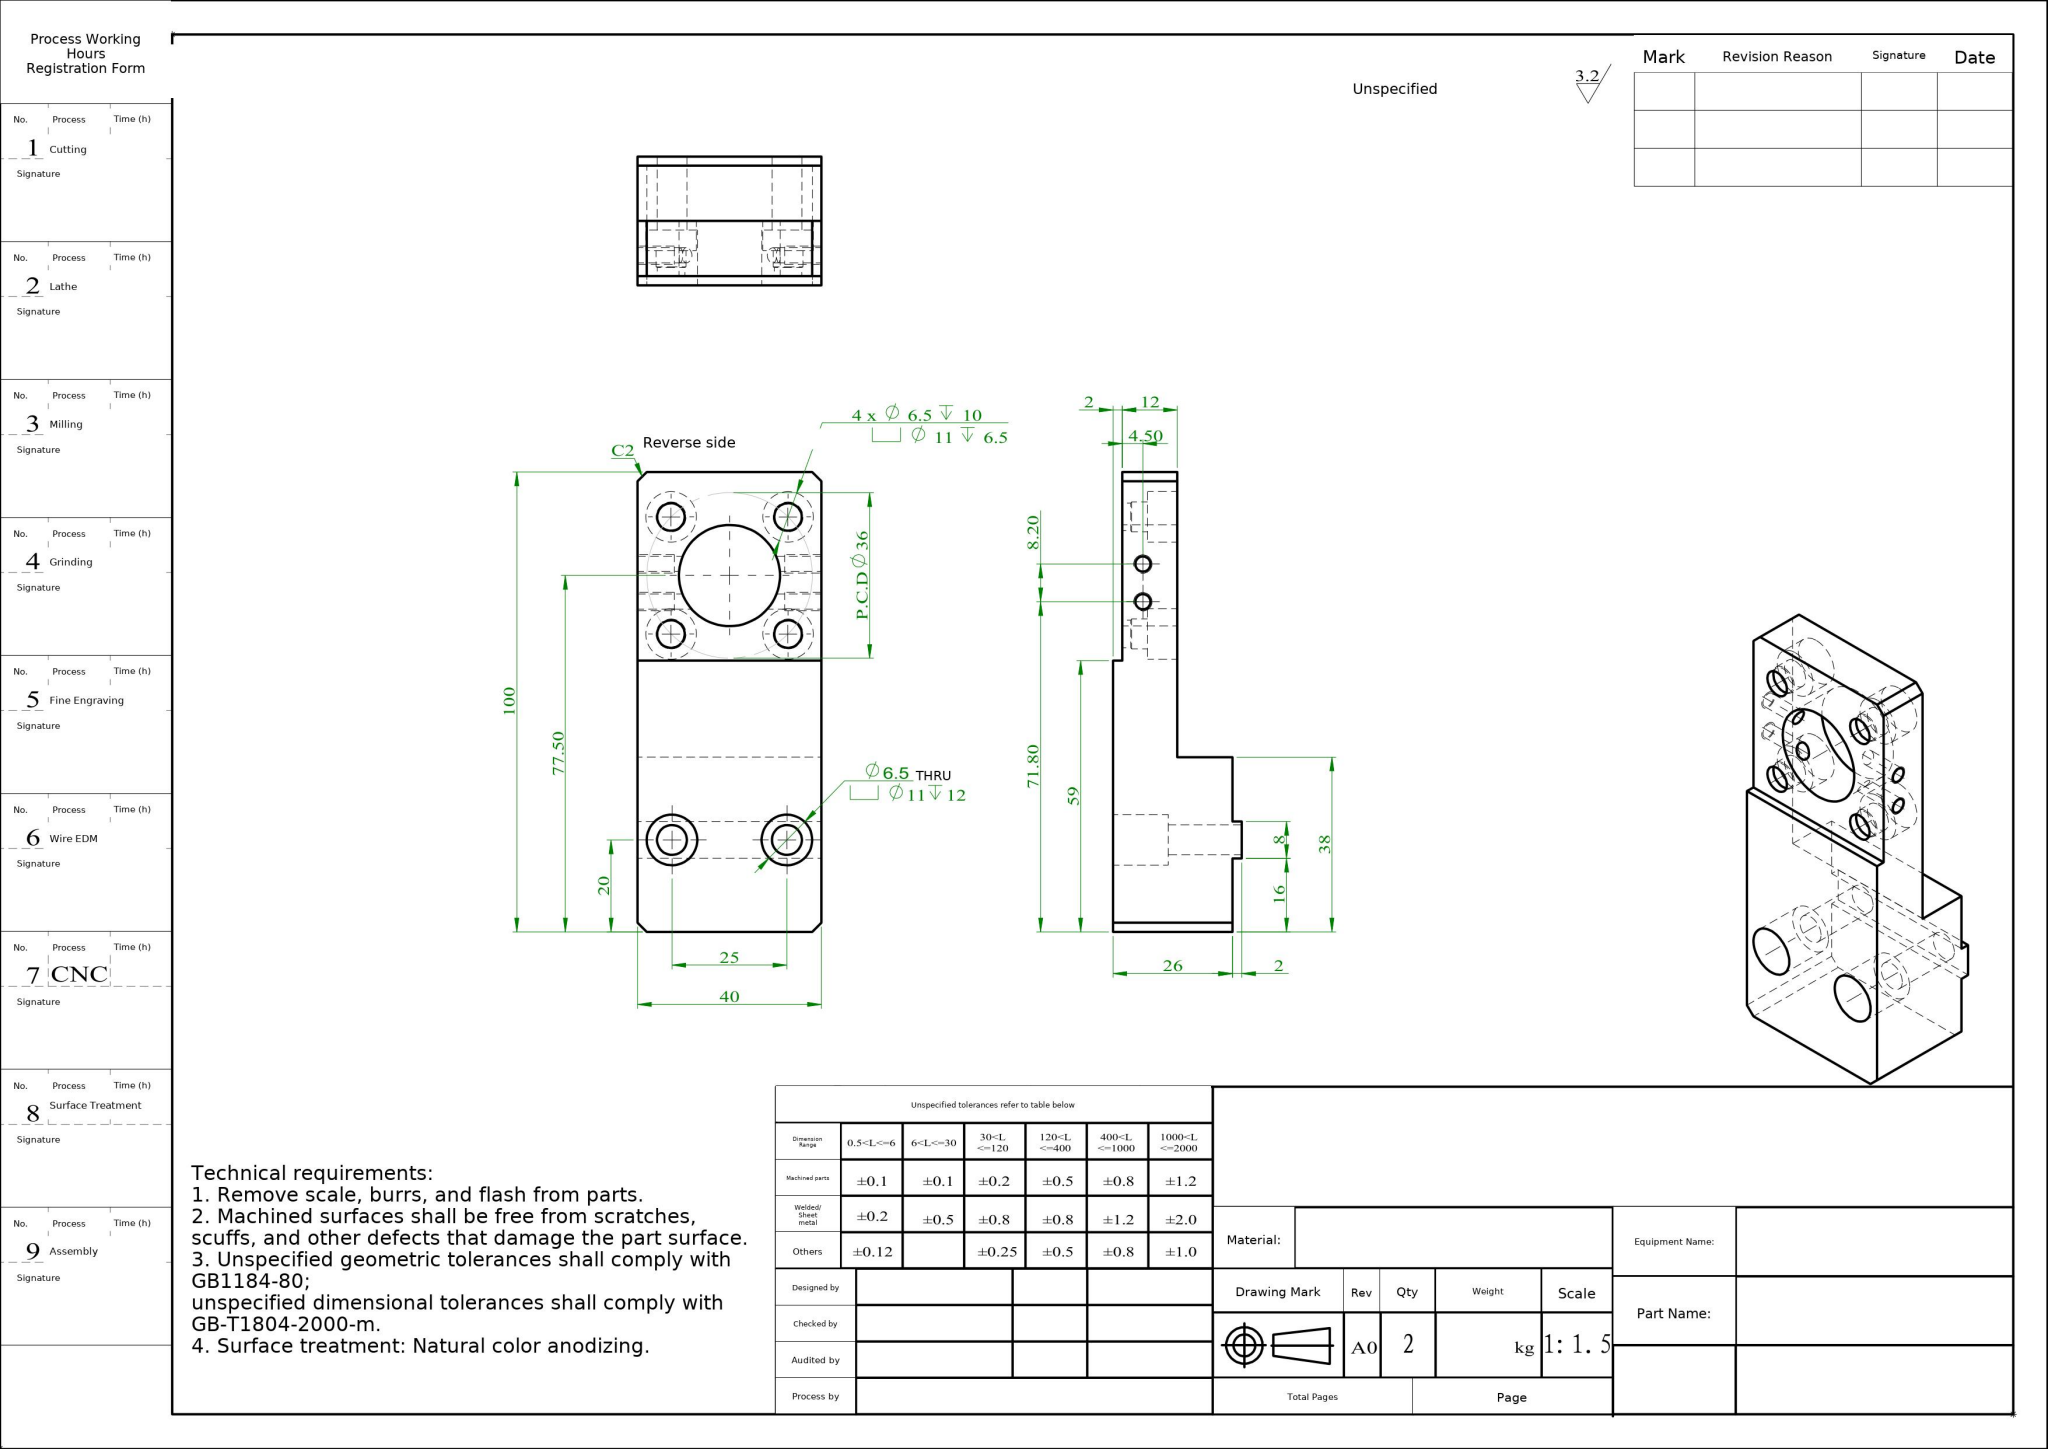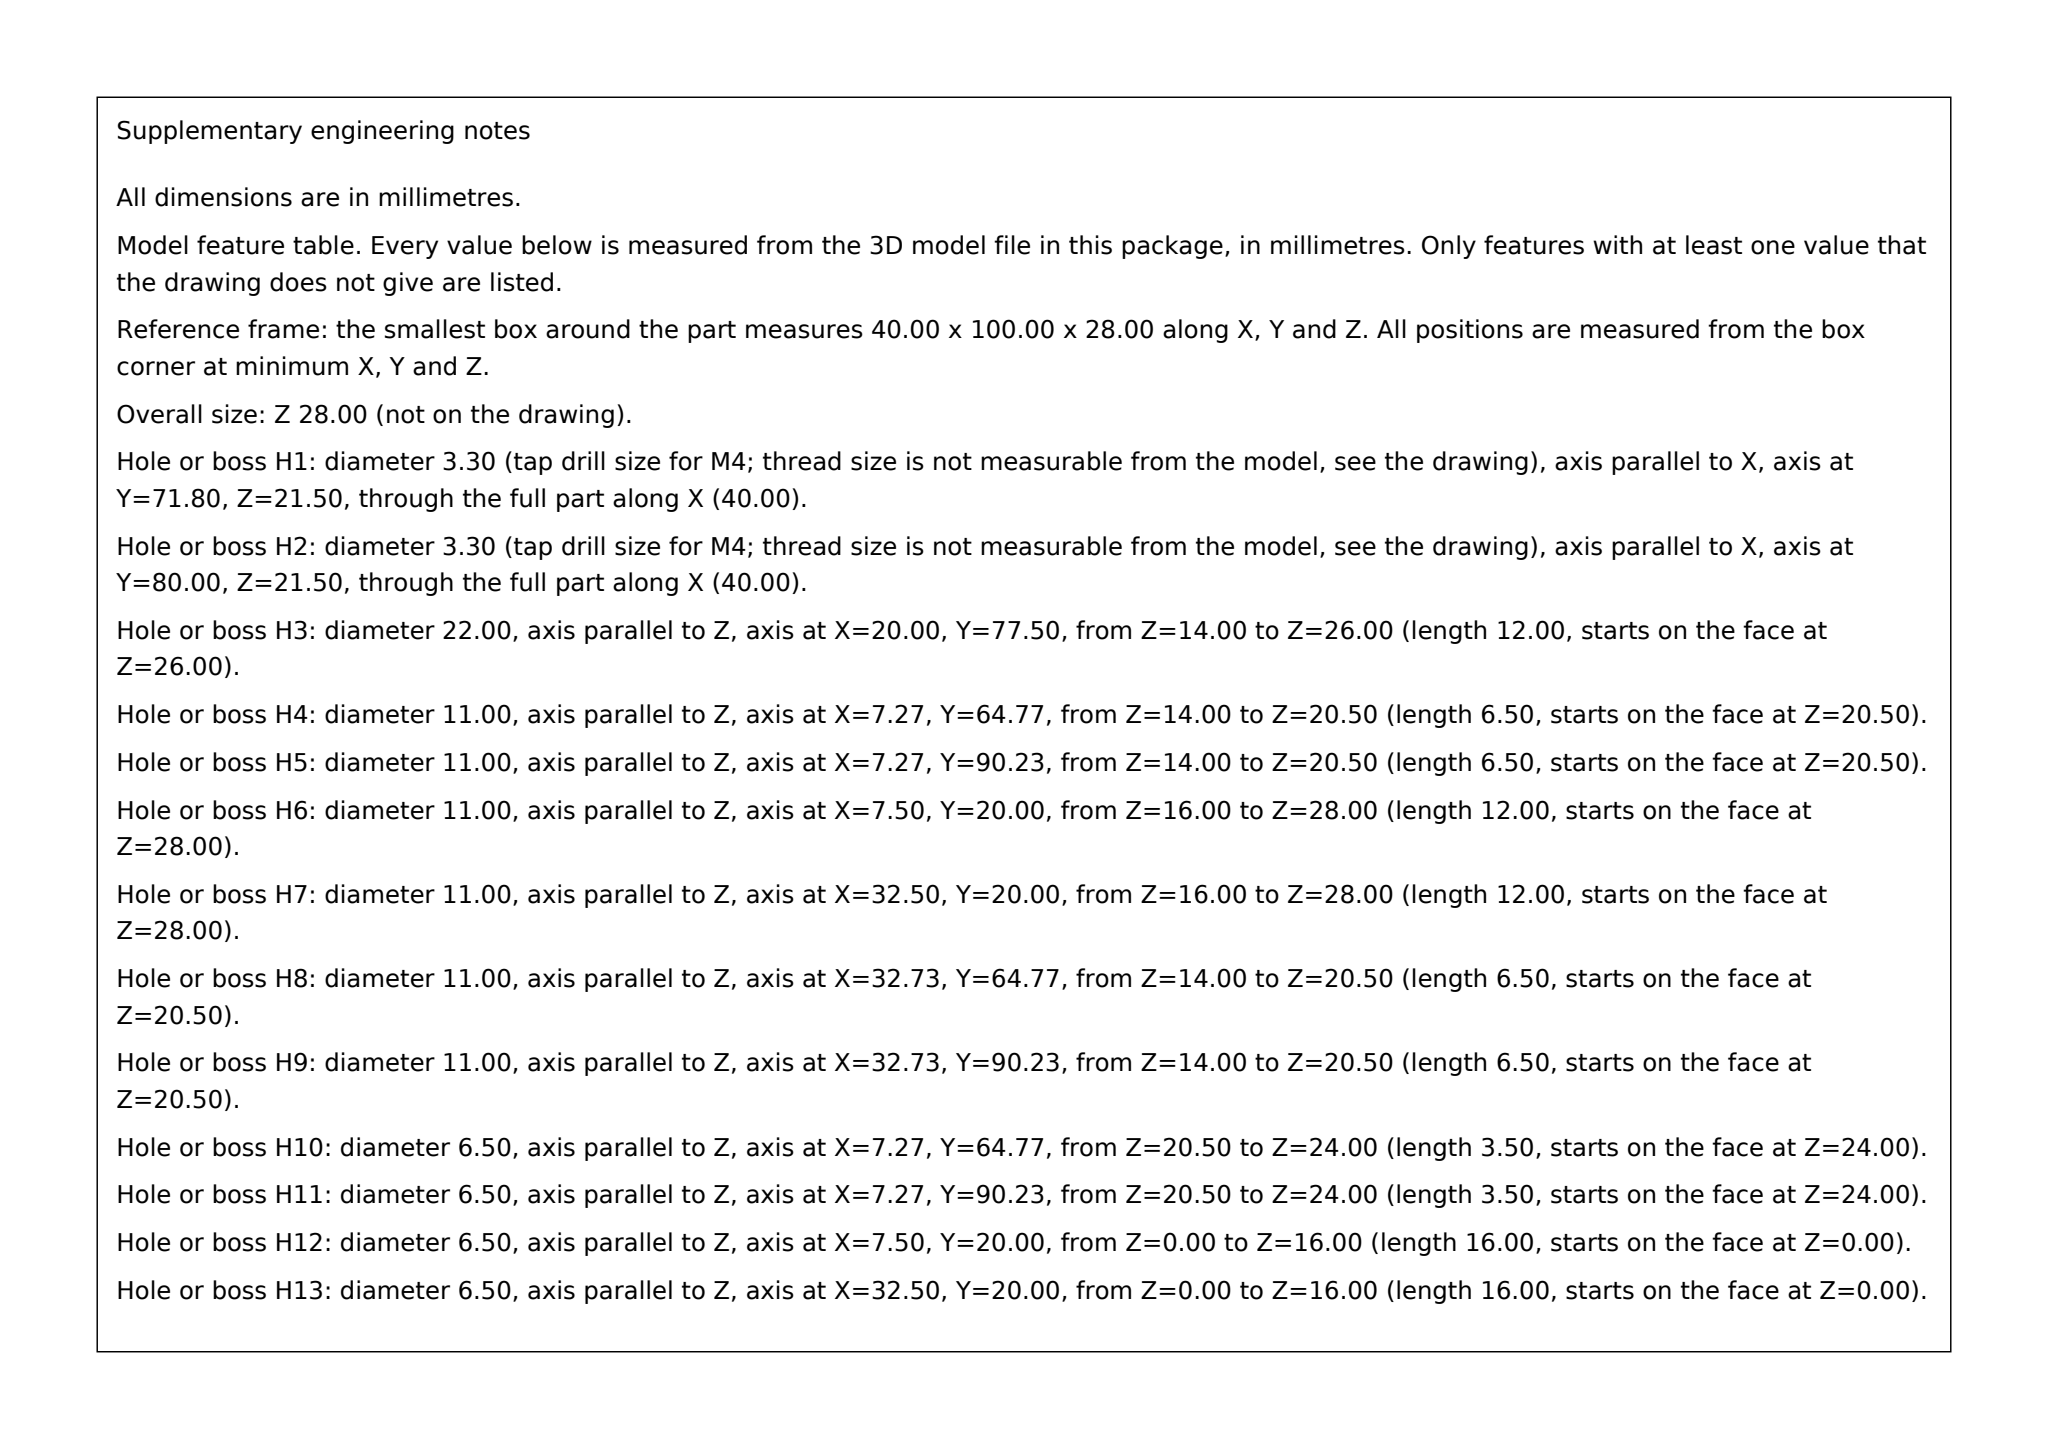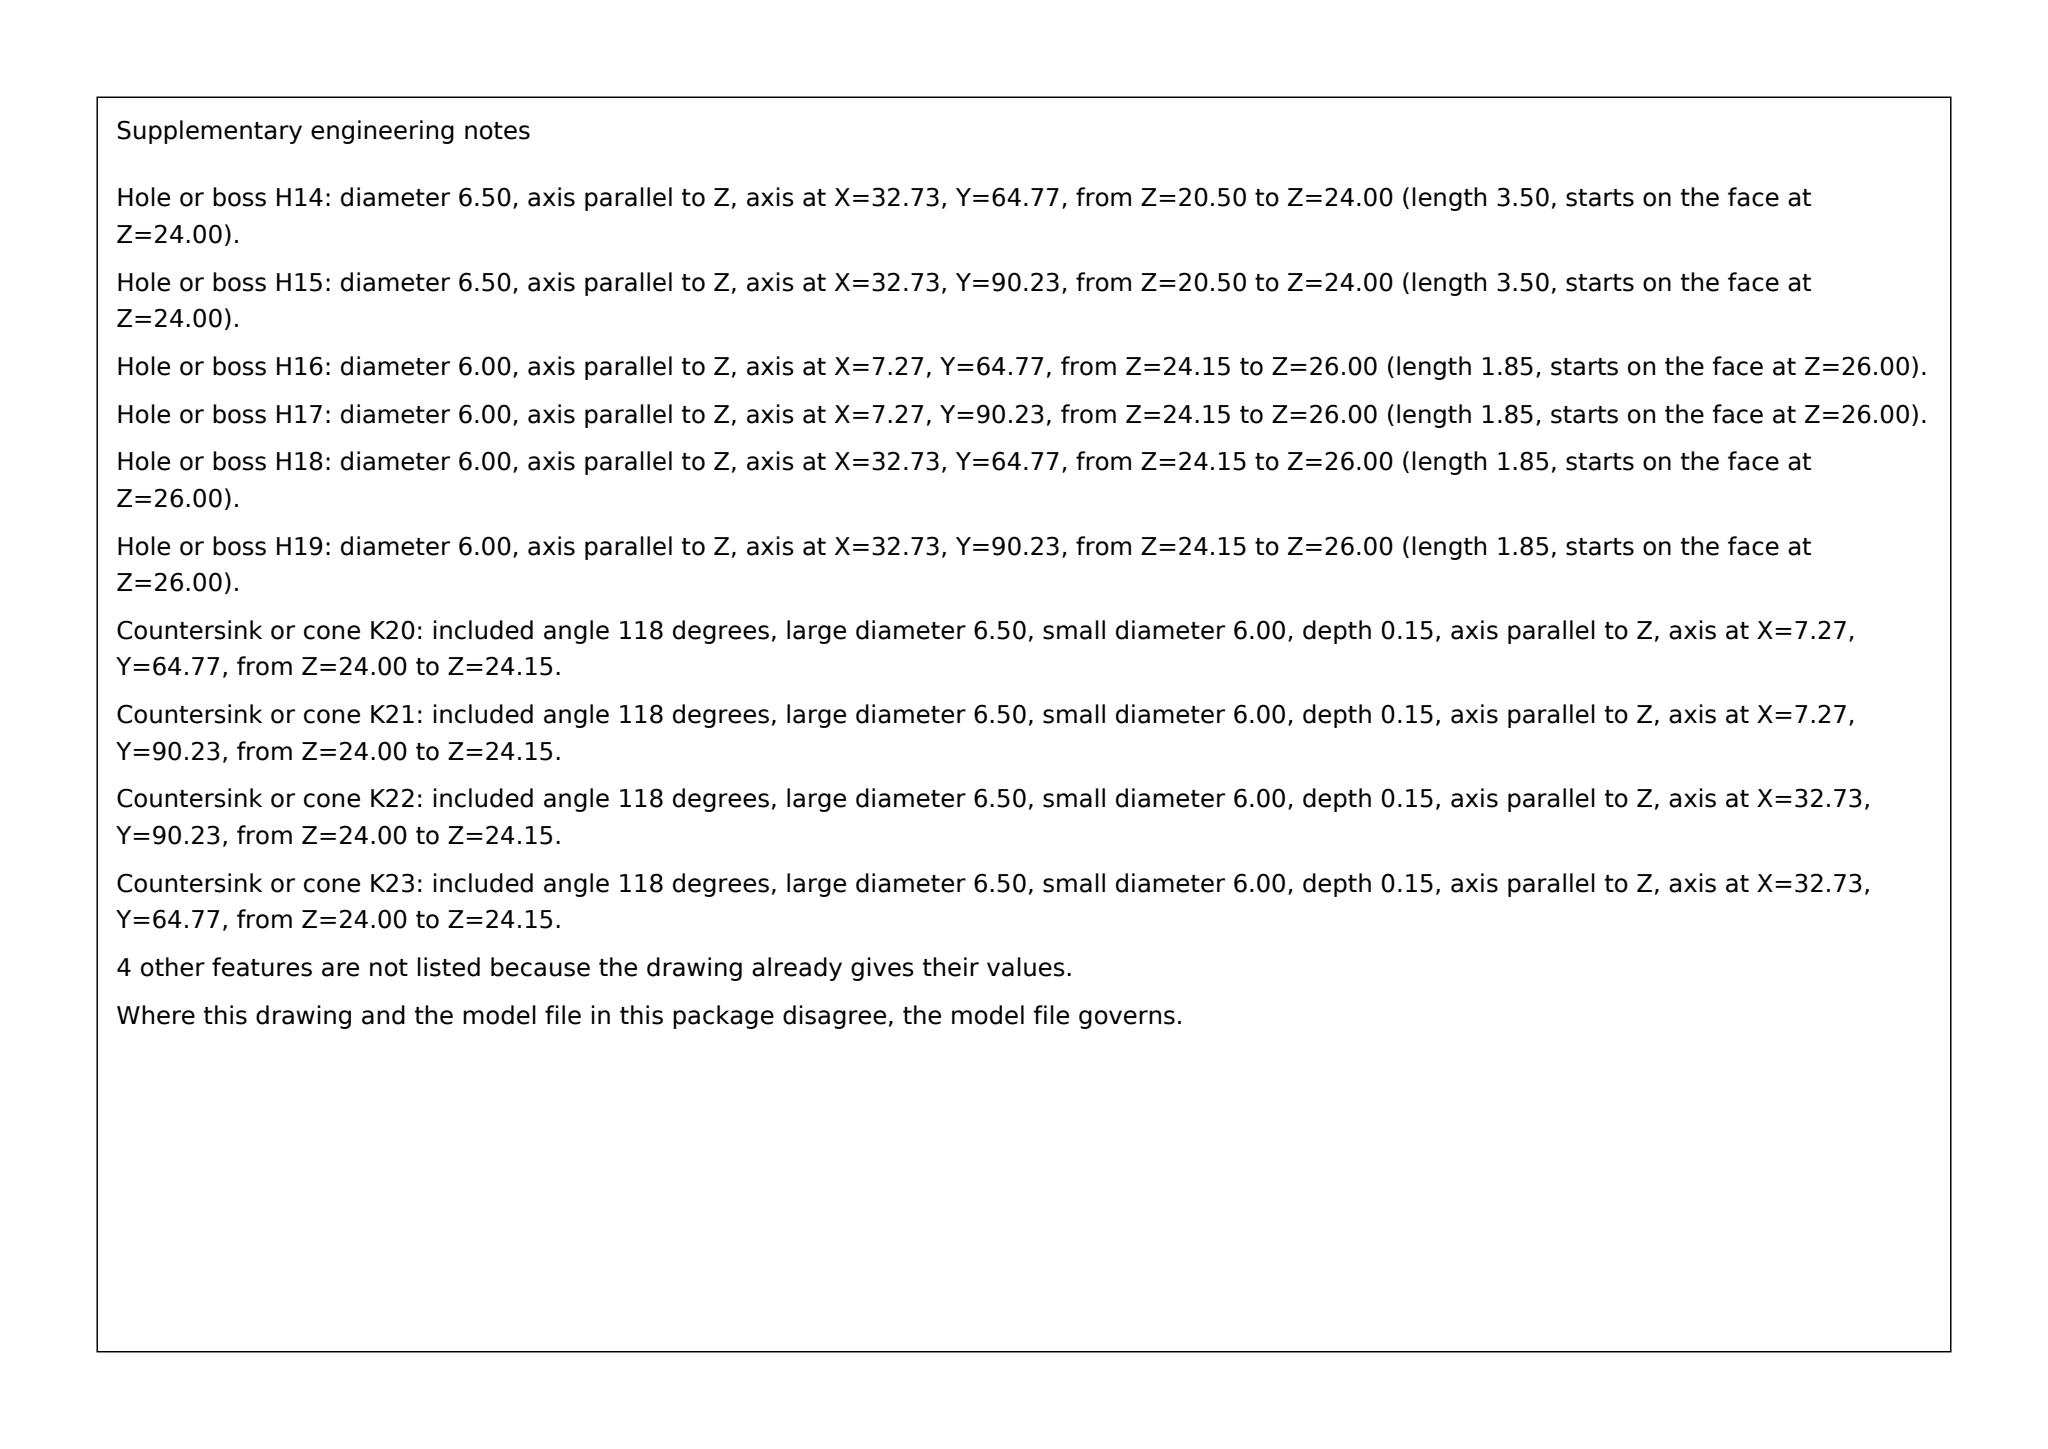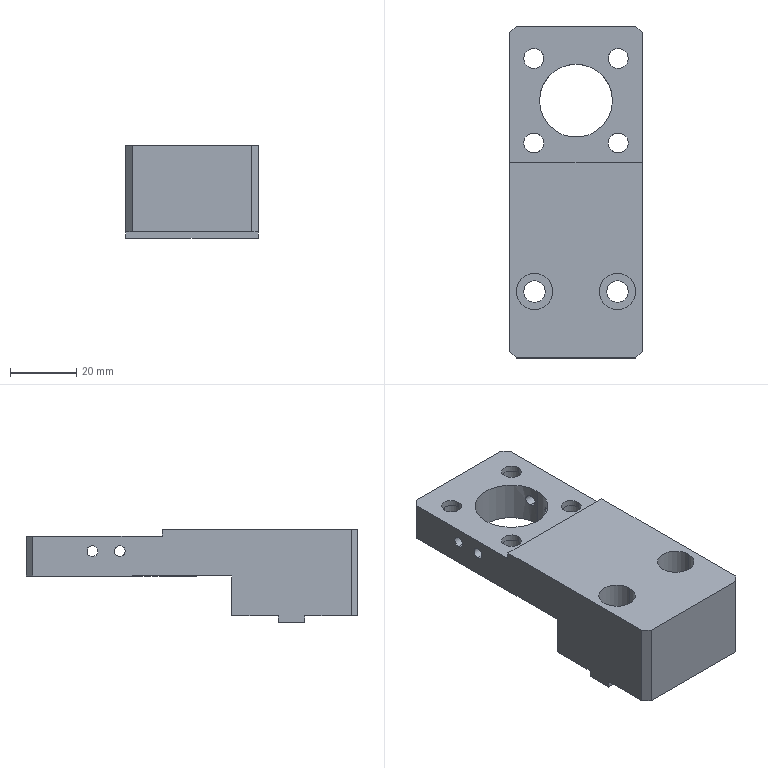Part | SolidWorks | mm | 1 solid | 74 faces | box 40 x 100 x 28 mm | volume 60039 mm3 | cylinder 42 | plane 24 | cone 8 | commonest cylinder face diameters 11 x12 6.5 x12 3.3 x8 6 x8 22 x2
build123d program:
from build123d import *

# Parameters (mm, degrees)
SKETCH1_W                                       = 40
SKETCH1_H                                       = 100
SKETCH1_R                                       = 3.25
EXTRUDE1_DEPTH                                  = 28
SKETCH2_R                                       = 5.5
EXTRUDE2_DEPTH                                  = 12
SKETCH3_W                                       = 14
SKETCH3_H                                       = 62
EXTRUDE3_DEPTH                                  = 60
SKETCH4_OUTSIDE_W                               = 64.256
SKETCH4_OUTSIDE_H                               = 124.256
SKETCH4_OUTSIDE_W_2                             = 40
SKETCH4_OUTSIDE_H_2                             = 8
EXTRUDE4_DEPTH                                  = 2
SKETCH5_R                                       = 11
SKETCH5_R_2                                     = 3
EXTRUDE5_DEPTH                                  = 112.283
CHAMFER1_SIZE                                   = 2
M4_TAPPED_HOLE1_AT_2_COUNT                      = 2
M4_TAPPED_HOLE1_AT_2_PITCH                      = 8.2
SKETCH12_W                                      = 40
SKETCH12_H                                      = 41
CUT_EXTRUDE1_DEPTH                              = 2
M6_HEX_SOCKET_HEAD_CAP_SCREW_CBORE4_D           = 6.5
M6_HEX_SOCKET_HEAD_CAP_SCREW_CBORE4_DEPTH       = 10
M6_HEX_SOCKET_HEAD_CAP_SCREW_CBORE4_CBORE_D     = 11
M6_HEX_SOCKET_HEAD_CAP_SCREW_CBORE4_CBORE_DEPTH = 6.5
M6_HEX_SOCKET_HEAD_CAP_SCREW_CBORE4_TIP         = 1.953


with BuildPart() as part:
    # Sketch1 → Extrude1 (new body)
    with BuildSketch(Plane.XY):
        with Locations((20, 50)):
            Rectangle(SKETCH1_W, SKETCH1_H)
        with Locations((7.5, 20)):
            Circle(SKETCH1_R, mode=Mode.SUBTRACT)
        with Locations((32.5, 20)):
            Circle(SKETCH1_R, mode=Mode.SUBTRACT)
    extrude(amount=EXTRUDE1_DEPTH)

    # Sketch2 → Extrude2 (cut)
    with BuildSketch(Plane.XY.offset(28)):
        with Locations((7.5, 20)):
            Circle(SKETCH2_R)
        with Locations((32.5, 20)):
            Circle(SKETCH2_R)
    extrude(amount=-EXTRUDE2_DEPTH, mode=Mode.SUBTRACT)

    # Sketch3 → Extrude3 (cut)
    with BuildSketch(Plane.ZY):
        with Locations((7, 69)):
            Rectangle(SKETCH3_W, SKETCH3_H)
    extrude(amount=-EXTRUDE3_DEPTH, mode=Mode.SUBTRACT)

    # Sketch4 outside → Extrude4 (cut)
    with BuildSketch(Plane(origin=(0, 0, 0), x_dir=(-1, 0, 0), z_dir=(0, 0, -1))):
        with Locations((-20, 50)):
            Rectangle(SKETCH4_OUTSIDE_W, SKETCH4_OUTSIDE_H)
        with Locations((-20, 20)):
            Rectangle(SKETCH4_OUTSIDE_W_2, SKETCH4_OUTSIDE_H_2, mode=Mode.SUBTRACT)
    extrude(amount=-EXTRUDE4_DEPTH, mode=Mode.SUBTRACT)

    # Sketch5 → Extrude5 (cut, through all)
    with BuildSketch(Plane.XY.offset(28)):
        with Locations((20, 77.5)):
            Circle(SKETCH5_R)
        with Locations((32.728, 90.228)):
            Circle(SKETCH5_R_2)
        with Locations((7.272, 90.228)):
            Circle(SKETCH5_R_2)
        with Locations((7.272, 64.772)):
            Circle(SKETCH5_R_2)
        with Locations((32.728, 64.772)):
            Circle(SKETCH5_R_2)
    extrude(amount=-EXTRUDE5_DEPTH, mode=Mode.SUBTRACT)

    # Chamfer1
    chamfer1_edges = [part.edges().sort_by_distance(p)[0] for p in [
        (0, 100, 21),
        (40, 100, 21),
        (40, 0, 15),
        (0, 0, 15),
    ]]
    chamfer(chamfer1_edges, length=CHAMFER1_SIZE)

    # Sketch9 → M4 Tapped Hole1 (revolve, cut)
    with BuildSketch(Plane(origin=(40, 80, 21.5), x_dir=(0, 0, -1), z_dir=(0, 1, 0))):
        Polygon((0, 0), (0, 12.991), (1.65, 12), (1.65, 0), align=None)
    m4_tapped_hole1 = revolve(axis=Axis((46.35, 80, 21.5), (-1, 0, 0)), mode=Mode.SUBTRACT)

    # M4 Tapped Hole1 at 2: M4 Tapped Hole1 ×2
    with Locations(*[(0, -i * M4_TAPPED_HOLE1_AT_2_PITCH, 0) for i in range(1, M4_TAPPED_HOLE1_AT_2_COUNT)]):
        add(m4_tapped_hole1, mode=Mode.SUBTRACT)

    # Mirror1: M4 Tapped Hole1 across plane
    add(m4_tapped_hole1.mirror(Plane(origin=(20, 0, 0), x_dir=(0, 0, 1), z_dir=(1, 0, 0))), mode=Mode.SUBTRACT)

    # Mirror1 copy 1 sketch → Mirror1 copy 1 (revolve, cut)
    with BuildSketch(Plane(origin=(0, 71.8, 21.5), x_dir=(0, 0, -1), z_dir=(0, 1, 0))):
        Polygon((0, 0), (0, -12.991), (1.65, -12), (1.65, 0), align=None)
    revolve(axis=Axis((-6.35, 71.8, 21.5), (-1, 0, 0)), mode=Mode.SUBTRACT)

    # Sketch12 → Cut-Extrude1 (cut)
    with BuildSketch(Plane.XY.offset(28)):
        with Locations((20, 79.5)):
            Rectangle(SKETCH12_W, SKETCH12_H)
    extrude(amount=-CUT_EXTRUDE1_DEPTH, mode=Mode.SUBTRACT)

    # M6 Hex Socket Head Cap Screw CBORE4
    with Locations(Plane(origin=(0, 0, 14), x_dir=(-1, 0, 0), z_dir=(0, 0, -1))):
        with Locations((-32.728, 90.228), (-7.272, 90.228), (-7.272, 64.772), (-32.728, 64.772)):
            CounterBoreHole(M6_HEX_SOCKET_HEAD_CAP_SCREW_CBORE4_D / 2, M6_HEX_SOCKET_HEAD_CAP_SCREW_CBORE4_CBORE_D / 2, M6_HEX_SOCKET_HEAD_CAP_SCREW_CBORE4_CBORE_DEPTH, depth=M6_HEX_SOCKET_HEAD_CAP_SCREW_CBORE4_DEPTH)
            with Locations((0, 0, -(M6_HEX_SOCKET_HEAD_CAP_SCREW_CBORE4_DEPTH + M6_HEX_SOCKET_HEAD_CAP_SCREW_CBORE4_TIP / 2))):  # 118° drill point
                Cone(0, M6_HEX_SOCKET_HEAD_CAP_SCREW_CBORE4_D / 2, M6_HEX_SOCKET_HEAD_CAP_SCREW_CBORE4_TIP, mode=Mode.SUBTRACT)


solid = part.part